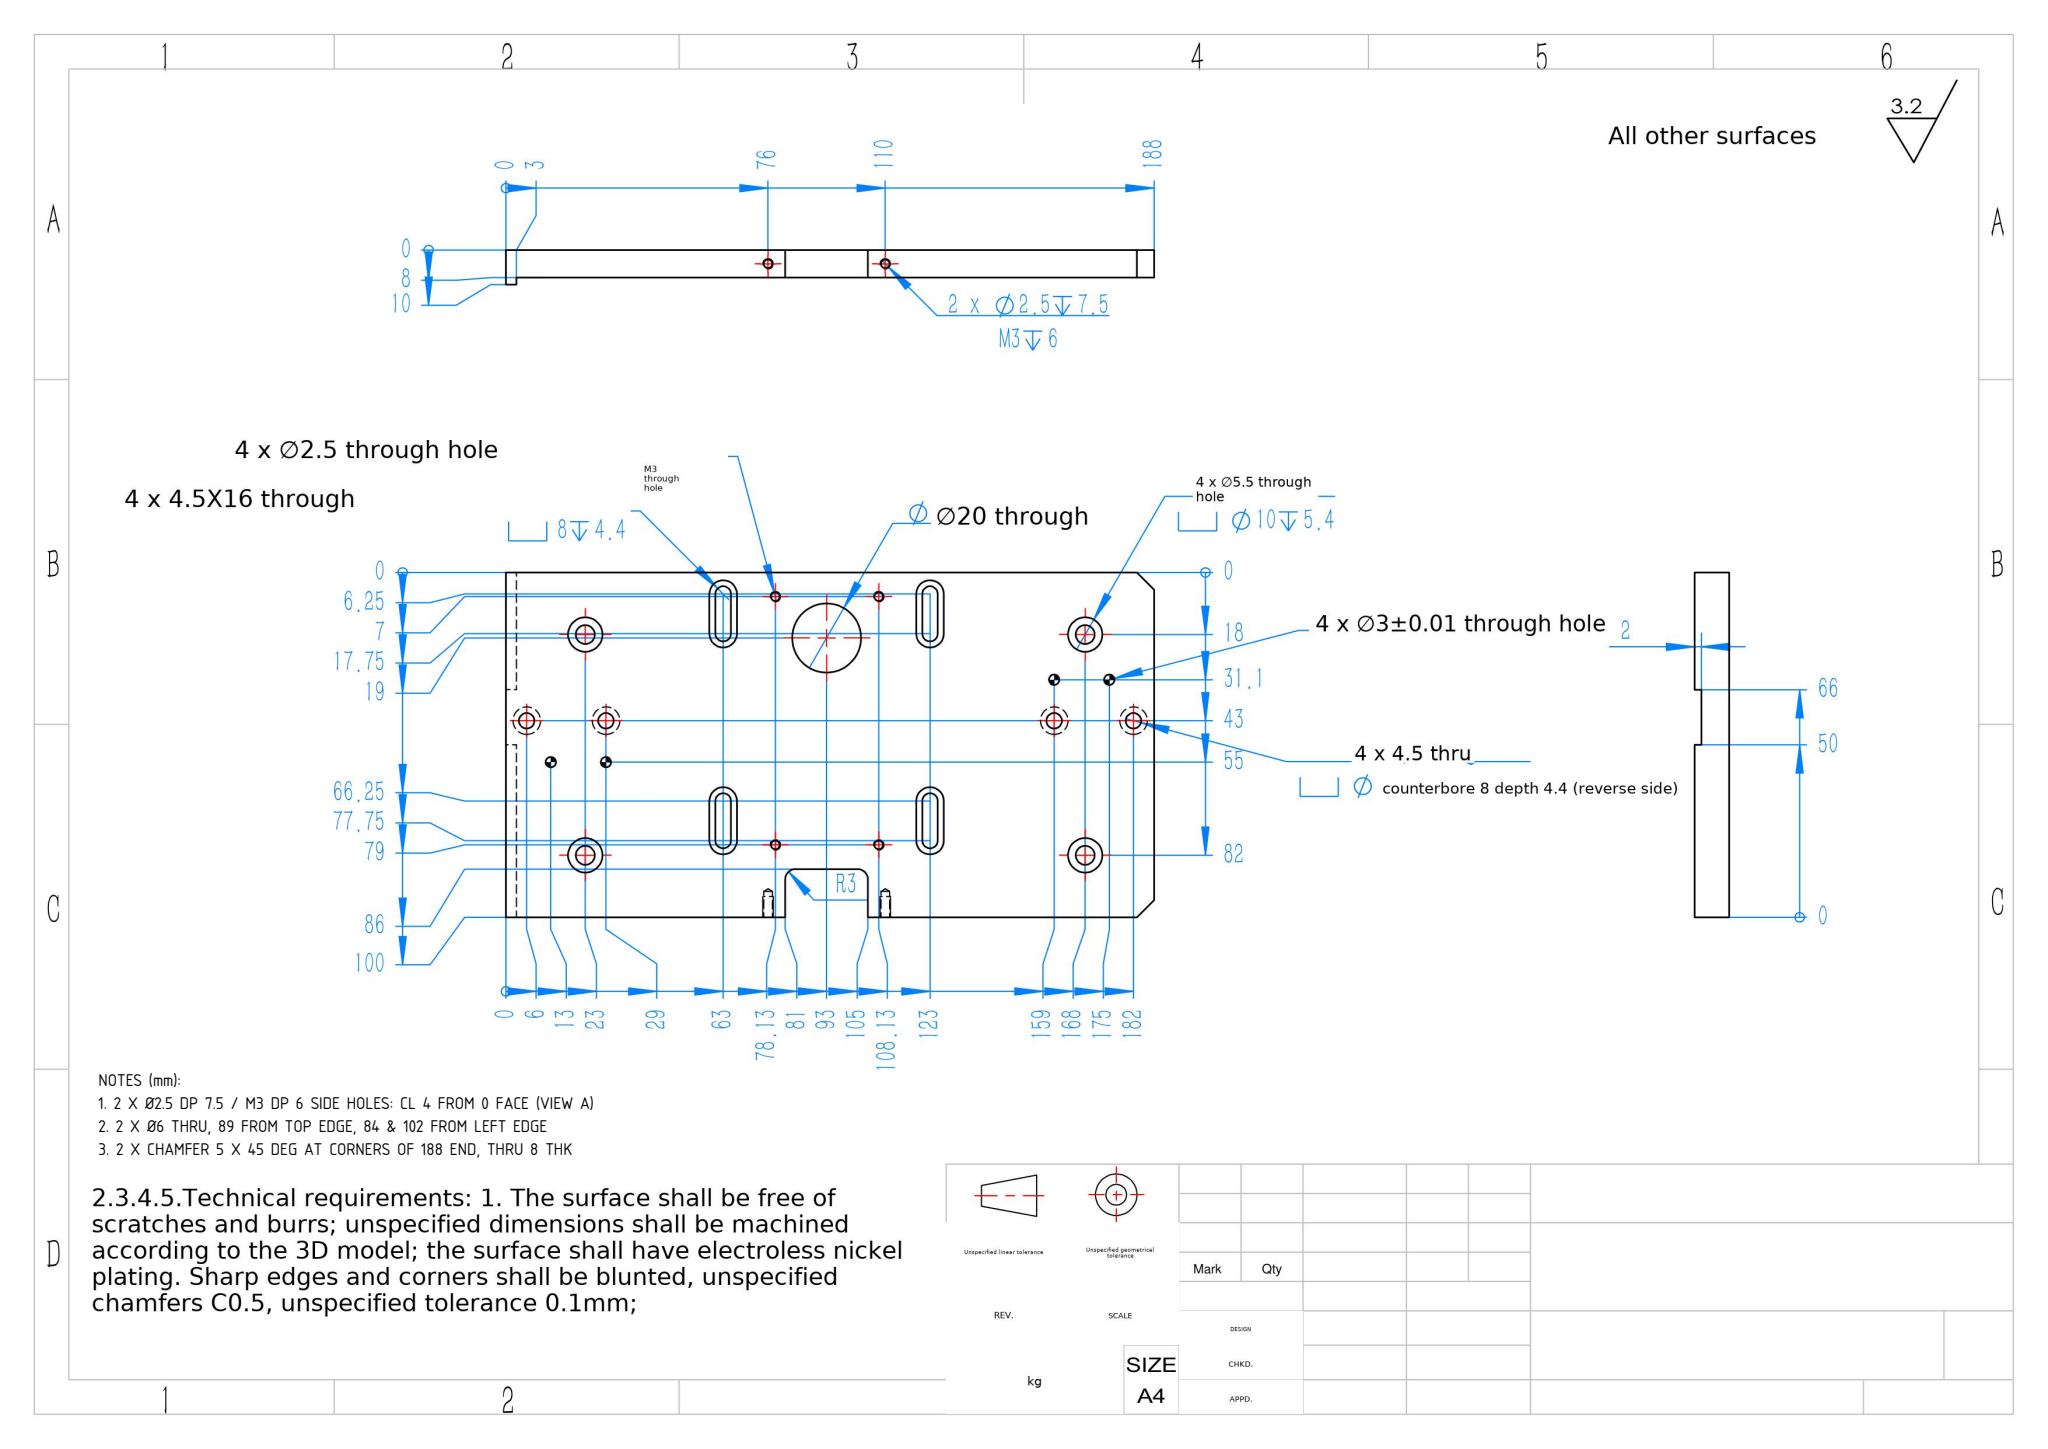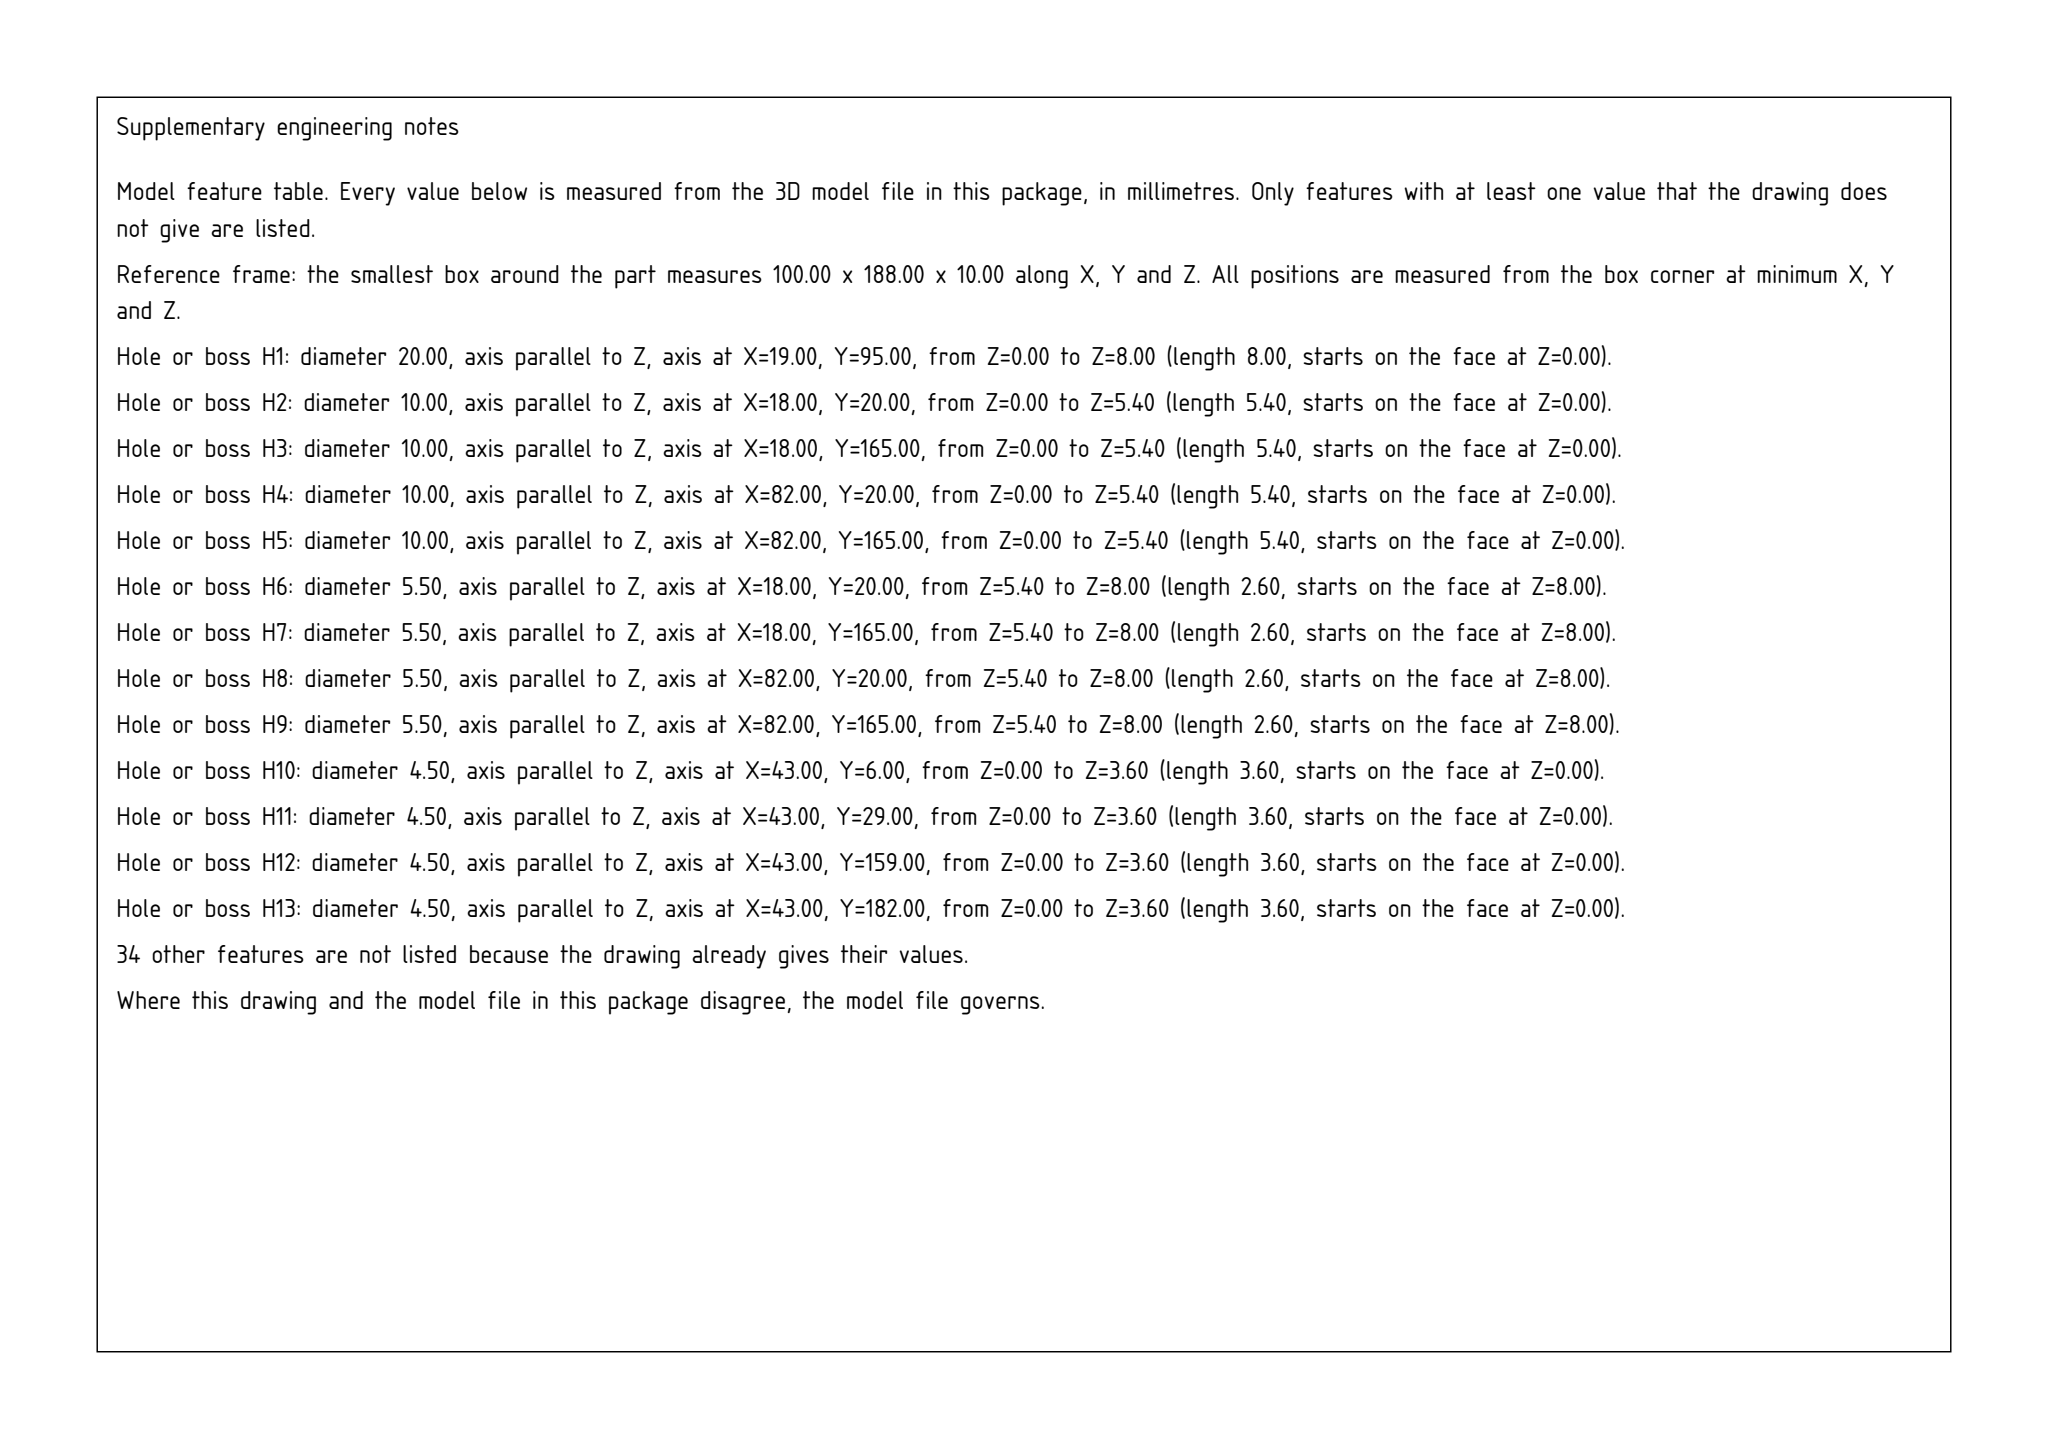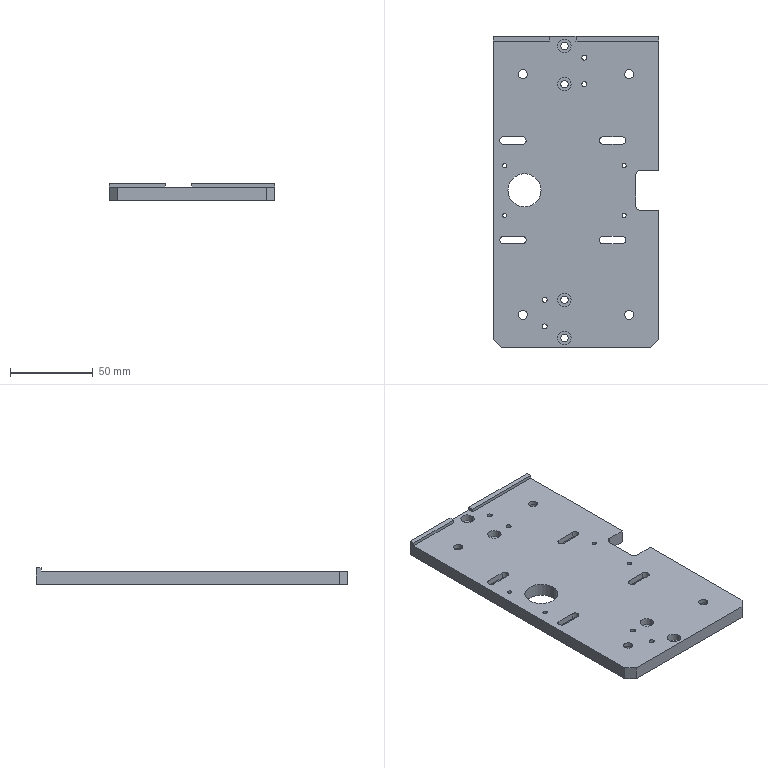Part | SolidWorks | mm | 1 solid | 130 faces | box 100 x 188 x 10 mm | volume 138539 mm3 | cylinder 80 | plane 46 | cone 4 | commonest cylinder face diameters 8 x20 4.5 x20 2.5 x12 3 x8 10 x8 5.5 x8 20 x2 6 x2
Drawing notes:
2 X Ø2.5 DP 7.5 / M3 DP 6 SIDE HOLES: CL 4 FROM 0 FACE (VIEW A) | from the solid: cylinders dia 2.5 axis x at [null,78,4] and [null,112,4], len 7.5 -> axis z=4.0 above z=0 datum face (z planes 0, 8, 10)
2 X Ø6 THRU, 89 FROM TOP EDGE, 84 & 102 FROM LEFT EDGE | from the solid: cyl dia 6.0 axis z, pos (x=89, y=86) and (x=89, y=104), len 8 = full plate thk; drawing vert = STEP x (89 from 0 top edge), drawing horiz = 188 - STEP y (84 and 102 from 0 left datum)
2 X CHAMFER 5 X 45 DEG AT CORNERS OF 188 END, THRU 8 THK | from the solid: inclined_planes: angle_to_xyz [45,45,90], bbox_from [0,0,0] and [95,0,0], size [5,5,8] - two 45 deg corner chamfers 5x5, full 8 mm thickness, at the y=0/188-length end corners (x=0 and x=100 edges)